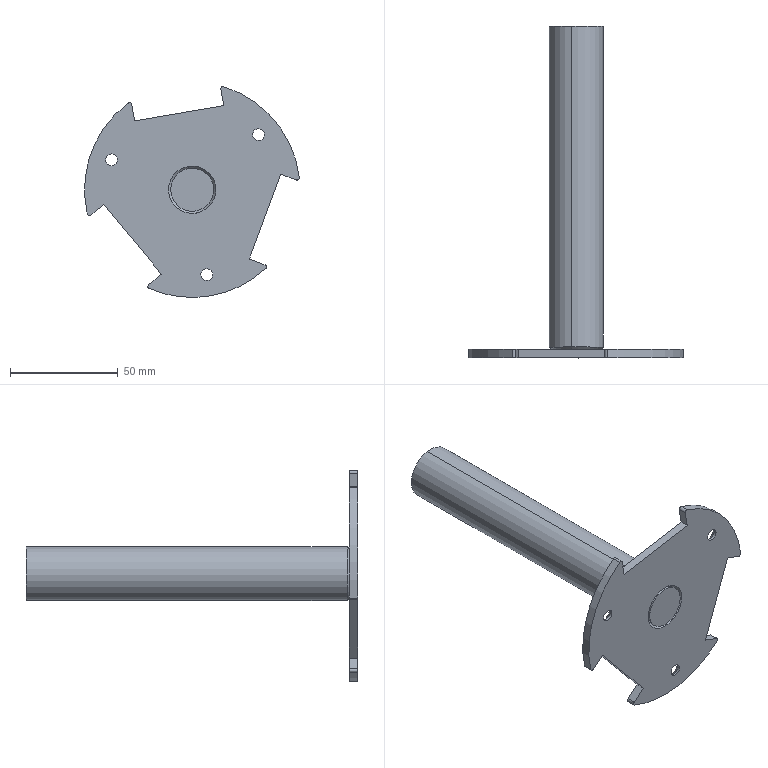Component | SolidWorks | 026A-20130717-1 | 3 solids | 53 faces | volume 96661 mm3 | cylinder 26 | plane 15 | cone 12 | commonest cylinder face diameters 2 x8 5.5 x6 20 x4 100 x4 8.5 x2 25 x2